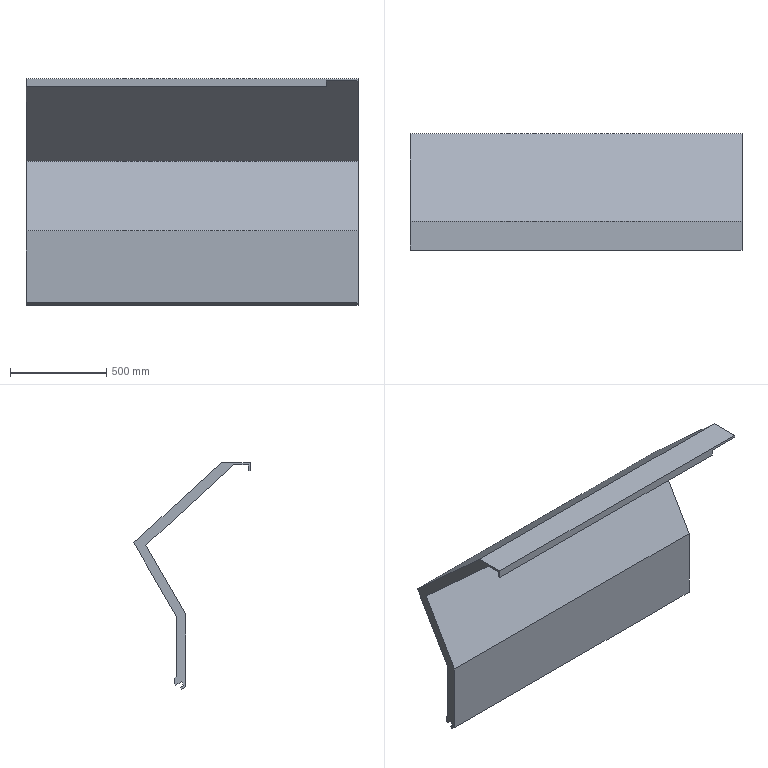Component | NX | SIM15_ABDECKUNG_OBEN_RECHTS | 1 solid | 26 faces | volume 125982613 mm3 | plane 26